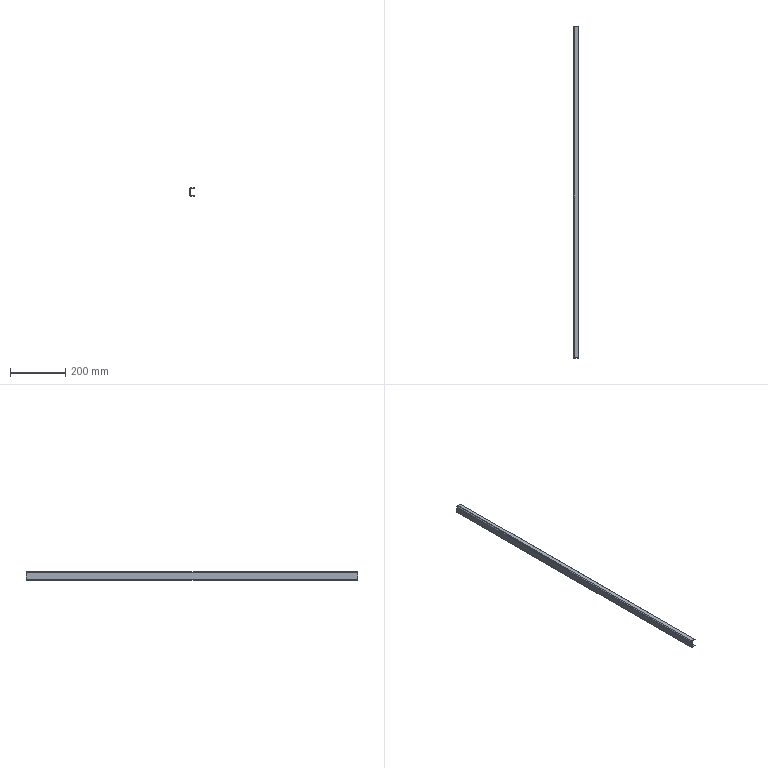Component | SolidWorks | MiddleTopCoverAssembly-1_TopCoverStiffener-1 | 1 solid | 30 faces | box 18 x 1200 x 30 mm | volume 142406 mm3 | plane 26 | cylinder 4 | commonest cylinder face diameters 8 x2 4 x2 | material Plain Carbon Steel
STEP:
#1=CARTESIAN_POINT('',(45.051,0.5334,82.479));
#2=VERTEX_POINT('',#1);
#3=CARTESIAN_POINT('',(45.051,0.5334,82.499));
#4=VERTEX_POINT('',#3);
#5=CARTESIAN_POINT('',(45.051,0.5334,82.42));
#6=DIRECTION('',(-0.,-0.,1.));
#7=VECTOR('',#6,39.37);
#8=LINE('',#5,#7);
#9=EDGE_CURVE('',#2,#4,#8,.T.);
#10=ORIENTED_EDGE('',*,*,#9,.F.);
#11=CARTESIAN_POINT('',(45.051,0.6201,82.479));
#12=VERTEX_POINT('',#11);
#13=CARTESIAN_POINT('',(45.051,47.778,82.479));
#14=DIRECTION('',(0.,1.,0.));
#15=VECTOR('',#14,39.37);
#16=LINE('',#13,#15);
#17=EDGE_CURVE('',#2,#12,#16,.T.);
#18=ORIENTED_EDGE('',*,*,#17,.T.);
#19=CARTESIAN_POINT('',(45.051,0.6201,82.42));
#20=VERTEX_POINT('',#19);
#21=CARTESIAN_POINT('',(45.051,0.6201,82.42));
#22=DIRECTION('',(0.,0.,-1.));
#23=VECTOR('',#22,39.37);
#24=LINE('',#21,#23);
#25=EDGE_CURVE('',#12,#20,#24,.T.);
#26=ORIENTED_EDGE('',*,*,#25,.T.);
#27=CARTESIAN_POINT('',(45.051,47.691,82.42));
#28=VERTEX_POINT('',#27);
#29=CARTESIAN_POINT('',(45.051,47.778,82.42));
#30=DIRECTION('',(-0.,-1.,-0.));
#31=VECTOR('',#30,39.37);
#32=LINE('',#29,#31);
#33=EDGE_CURVE('',#28,#20,#32,.T.);
#34=ORIENTED_EDGE('',*,*,#33,.F.);
#35=CARTESIAN_POINT('',(45.051,47.691,82.479));
#36=VERTEX_POINT('',#35);
#37=CARTESIAN_POINT('',(45.051,47.691,82.42));
#38=DIRECTION('',(-0.,-0.,1.));
#39=VECTOR('',#38,39.37);
#40=LINE('',#37,#39);
#41=EDGE_CURVE('',#28,#36,#40,.T.);
#42=ORIENTED_EDGE('',*,*,#41,.T.);
#43=CARTESIAN_POINT('',(45.051,47.778,82.479));
#44=VERTEX_POINT('',#43);
#45=CARTESIAN_POINT('',(45.051,47.778,82.479));
#46=DIRECTION('',(0.,1.,0.));
#47=VECTOR('',#46,39.37);
#48=LINE('',#45,#47);
#49=EDGE_CURVE('',#36,#44,#48,.T.);
#50=ORIENTED_EDGE('',*,*,#49,.T.);
#51=CARTESIAN_POINT('',(45.051,47.778,82.499));
#52=VERTEX_POINT('',#51);
#53=CARTESIAN_POINT('',(45.051,47.778,82.42));
#54=DIRECTION('',(-0.,-0.,1.));
#55=VECTOR('',#54,39.37);
#56=LINE('',#53,#55);
#57=EDGE_CURVE('',#44,#52,#56,.T.);
#58=ORIENTED_EDGE('',*,*,#57,.T.);
#59=CARTESIAN_POINT('',(45.051,47.778,82.499));
#60=DIRECTION('',(-0.,-1.,-0.));
#61=VECTOR('',#60,39.37);
#62=LINE('',#59,#61);
#63=EDGE_CURVE('',#52,#4,#62,.T.);
#64=ORIENTED_EDGE('',*,*,#63,.T.);
#65=EDGE_LOOP('',(#10,#18,#26,#34,#42,#50,#58,#64));
#66=FACE_OUTER_BOUND('',#65,.T.);
#67=CARTESIAN_POINT('',(45.051,47.778,82.42));
#68=DIRECTION('',(1.,-0.,-0.));
#69=DIRECTION('',(0.,0.,-1.));
#70=AXIS2_PLACEMENT_3D('',#67,#68,#69);
#71=PLANE('',#70);
#72=ADVANCED_FACE('',(#66),#71,.T.);
#73=CARTESIAN_POINT('',(45.051,0.6201,83.602));
#74=VERTEX_POINT('',#73);
#75=CARTESIAN_POINT('',(45.051,0.6201,83.543));
#76=VERTEX_POINT('',#75);
#77=CARTESIAN_POINT('',(45.051,0.6201,83.523));
#78=DIRECTION('',(0.,0.,-1.));
#79=VECTOR('',#78,39.37);
#80=LINE('',#77,#79);
#81=EDGE_CURVE('',#74,#76,#80,.T.);
#82=ORIENTED_EDGE('',*,*,#81,.T.);
#83=CARTESIAN_POINT('',(45.051,0.5334,83.543));
#84=VERTEX_POINT('',#83);
#85=CARTESIAN_POINT('',(45.051,47.778,83.543));
#86=DIRECTION('',(-0.,-1.,-0.));
#87=VECTOR('',#86,39.37);
#88=LINE('',#85,#87);
#89=EDGE_CURVE('',#76,#84,#88,.T.);
#90=ORIENTED_EDGE('',*,*,#89,.T.);
#91=CARTESIAN_POINT('',(45.051,0.5334,83.523));
#92=VERTEX_POINT('',#91);
#93=CARTESIAN_POINT('',(45.051,0.5334,83.523));
#94=DIRECTION('',(-0.,-0.,1.));
#95=VECTOR('',#94,39.37);
#96=LINE('',#93,#95);
#97=EDGE_CURVE('',#92,#84,#96,.T.);
#98=ORIENTED_EDGE('',*,*,#97,.F.);
#99=CARTESIAN_POINT('',(45.051,47.778,83.523));
#100=VERTEX_POINT('',#99);
#101=CARTESIAN_POINT('',(45.051,47.778,83.523));
#102=DIRECTION('',(-0.,-1.,-0.));
#103=VECTOR('',#102,39.37);
#104=LINE('',#101,#103);
#105=EDGE_CURVE('',#100,#92,#104,.T.);
#106=ORIENTED_EDGE('',*,*,#105,.F.);
#107=CARTESIAN_POINT('',(45.051,47.778,83.543));
#108=VERTEX_POINT('',#107);
#109=CARTESIAN_POINT('',(45.051,47.778,83.523));
#110=DIRECTION('',(-0.,-0.,1.));
#111=VECTOR('',#110,39.37);
#112=LINE('',#109,#111);
#113=EDGE_CURVE('',#100,#108,#112,.T.);
#114=ORIENTED_EDGE('',*,*,#113,.T.);
#115=CARTESIAN_POINT('',(45.051,47.691,83.543));
#116=VERTEX_POINT('',#115);
#117=CARTESIAN_POINT('',(45.051,47.778,83.543));
#118=DIRECTION('',(-0.,-1.,-0.));
#119=VECTOR('',#118,39.37);
#120=LINE('',#117,#119);
#121=EDGE_CURVE('',#108,#116,#120,.T.);
#122=ORIENTED_EDGE('',*,*,#121,.T.);
#123=CARTESIAN_POINT('',(45.051,47.691,83.602));
#124=VERTEX_POINT('',#123);
#125=CARTESIAN_POINT('',(45.051,47.691,83.523));
#126=DIRECTION('',(-0.,-0.,1.));
#127=VECTOR('',#126,39.37);
#128=LINE('',#125,#127);
#129=EDGE_CURVE('',#116,#124,#128,.T.);
#130=ORIENTED_EDGE('',*,*,#129,.T.);
#131=CARTESIAN_POINT('',(45.051,47.778,83.602));
#132=DIRECTION('',(-0.,-1.,-0.));
#133=VECTOR('',#132,39.37);
#134=LINE('',#131,#133);
#135=EDGE_CURVE('',#124,#74,#134,.T.);
#136=ORIENTED_EDGE('',*,*,#135,.T.);
#137=EDGE_LOOP('',(#82,#90,#98,#106,#114,#122,#130,#136));
#138=FACE_OUTER_BOUND('',#137,.T.);
#139=CARTESIAN_POINT('',(45.051,47.778,83.523));
#140=DIRECTION('',(1.,-0.,-0.));
#141=DIRECTION('',(-0.,-1.,-0.));
#142=AXIS2_PLACEMENT_3D('',#139,#140,#141);
#143=PLANE('',#142);
#144=ADVANCED_FACE('',(#138),#143,.T.);
#145=CARTESIAN_POINT('',(44.499,47.778,83.543));
#146=VERTEX_POINT('',#145);
#147=CARTESIAN_POINT('',(44.377,47.778,83.543));
#148=VERTEX_POINT('',#147);
#149=CARTESIAN_POINT('',(44.342,47.778,83.543));
#150=DIRECTION('',(-1.,0.,0.));
#151=VECTOR('',#150,39.37);
#152=LINE('',#149,#151);
#153=EDGE_CURVE('',#146,#148,#152,.T.);
#154=ORIENTED_EDGE('',*,*,#153,.F.);
#155=CARTESIAN_POINT('',(44.499,47.778,83.523));
#156=VERTEX_POINT('',#155);
#157=CARTESIAN_POINT('',(44.499,47.778,83.523));
#158=DIRECTION('',(-0.,-0.,1.));
#159=VECTOR('',#158,39.37);
#160=LINE('',#157,#159);
#161=EDGE_CURVE('',#156,#146,#160,.T.);
#162=ORIENTED_EDGE('',*,*,#161,.F.);
#163=CARTESIAN_POINT('',(44.421,47.778,83.444));
#164=VERTEX_POINT('',#163);
#165=CARTESIAN_POINT('',(44.499,47.778,83.444));
#166=DIRECTION('',(-0.,-1.,-0.));
#167=DIRECTION('',(0.,0.,-1.));
#168=AXIS2_PLACEMENT_3D('',#165,#166,#167);
#169=CIRCLE('',#168,0.07874);
#170=EDGE_CURVE('',#156,#164,#169,.T.);
#171=ORIENTED_EDGE('',*,*,#170,.T.);
#172=CARTESIAN_POINT('',(44.342,47.778,83.444));
#173=VERTEX_POINT('',#172);
#174=CARTESIAN_POINT('',(44.342,47.778,83.444));
#175=DIRECTION('',(1.,-0.,-0.));
#176=VECTOR('',#175,39.37);
#177=LINE('',#174,#176);
#178=EDGE_CURVE('',#173,#164,#177,.T.);
#179=ORIENTED_EDGE('',*,*,#178,.F.);
#180=CARTESIAN_POINT('',(44.499,47.778,83.444));
#181=DIRECTION('',(-0.,-1.,-0.));
#182=DIRECTION('',(0.,0.,-1.));
#183=AXIS2_PLACEMENT_3D('',#180,#181,#182);
#184=CIRCLE('',#183,0.1575);
#185=EDGE_CURVE('',#148,#173,#184,.T.);
#186=ORIENTED_EDGE('',*,*,#185,.F.);
#187=EDGE_LOOP('',(#154,#162,#171,#179,#186));
#188=FACE_OUTER_BOUND('',#187,.T.);
#189=CARTESIAN_POINT('',(44.342,47.778,83.444));
#190=DIRECTION('',(0.,1.,0.));
#191=DIRECTION('',(0.,0.,-1.));
#192=AXIS2_PLACEMENT_3D('',#189,#190,#191);
#193=PLANE('',#192);
#194=ADVANCED_FACE('',(#188),#193,.T.);
#195=CARTESIAN_POINT('',(44.342,47.778,82.578));
#196=VERTEX_POINT('',#195);
#197=CARTESIAN_POINT('',(44.342,47.778,83.602));
#198=DIRECTION('',(0.,0.,-1.));
#199=VECTOR('',#198,39.37);
#200=LINE('',#197,#199);
#201=EDGE_CURVE('',#173,#196,#200,.T.);
#202=ORIENTED_EDGE('',*,*,#201,.F.);
#203=ORIENTED_EDGE('',*,*,#178,.T.);
#204=CARTESIAN_POINT('',(44.421,47.778,82.578));
#205=VERTEX_POINT('',#204);
#206=CARTESIAN_POINT('',(44.421,47.778,83.602));
#207=DIRECTION('',(0.,0.,-1.));
#208=VECTOR('',#207,39.37);
#209=LINE('',#206,#208);
#210=EDGE_CURVE('',#164,#205,#209,.T.);
#211=ORIENTED_EDGE('',*,*,#210,.T.);
#212=CARTESIAN_POINT('',(44.421,47.778,82.578));
#213=DIRECTION('',(-1.,0.,0.));
#214=VECTOR('',#213,39.37);
#215=LINE('',#212,#214);
#216=EDGE_CURVE('',#205,#196,#215,.T.);
#217=ORIENTED_EDGE('',*,*,#216,.T.);
#218=EDGE_LOOP('',(#202,#203,#211,#217));
#219=FACE_OUTER_BOUND('',#218,.T.);
#220=CARTESIAN_POINT('',(44.499,47.778,83.523));
#221=DIRECTION('',(0.,1.,0.));
#222=DIRECTION('',(0.,0.,-1.));
#223=AXIS2_PLACEMENT_3D('',#220,#221,#222);
#224=PLANE('',#223);
#225=ADVANCED_FACE('',(#219),#224,.T.);
#226=CARTESIAN_POINT('',(44.377,0.5334,83.543));
#227=VERTEX_POINT('',#226);
#228=CARTESIAN_POINT('',(44.499,0.5334,83.543));
#229=VERTEX_POINT('',#228);
#230=CARTESIAN_POINT('',(44.499,0.5334,83.543));
#231=DIRECTION('',(1.,-0.,-0.));
#232=VECTOR('',#231,39.37);
#233=LINE('',#230,#232);
#234=EDGE_CURVE('',#227,#229,#233,.T.);
#235=ORIENTED_EDGE('',*,*,#234,.F.);
#236=CARTESIAN_POINT('',(44.342,0.5334,83.444));
#237=VERTEX_POINT('',#236);
#238=CARTESIAN_POINT('',(44.499,0.5334,83.444));
#239=DIRECTION('',(-0.,-1.,-0.));
#240=DIRECTION('',(0.,0.,-1.));
#241=AXIS2_PLACEMENT_3D('',#238,#239,#240);
#242=CIRCLE('',#241,0.1575);
#243=EDGE_CURVE('',#227,#237,#242,.T.);
#244=ORIENTED_EDGE('',*,*,#243,.T.);
#245=CARTESIAN_POINT('',(44.421,0.5334,83.444));
#246=VERTEX_POINT('',#245);
#247=CARTESIAN_POINT('',(44.421,0.5334,83.444));
#248=DIRECTION('',(-1.,0.,0.));
#249=VECTOR('',#248,39.37);
#250=LINE('',#247,#249);
#251=EDGE_CURVE('',#246,#237,#250,.T.);
#252=ORIENTED_EDGE('',*,*,#251,.F.);
#253=CARTESIAN_POINT('',(44.499,0.5334,83.523));
#254=VERTEX_POINT('',#253);
#255=CARTESIAN_POINT('',(44.499,0.5334,83.444));
#256=DIRECTION('',(-0.,-1.,-0.));
#257=DIRECTION('',(0.,0.,-1.));
#258=AXIS2_PLACEMENT_3D('',#255,#256,#257);
#259=CIRCLE('',#258,0.07874);
#260=EDGE_CURVE('',#254,#246,#259,.T.);
#261=ORIENTED_EDGE('',*,*,#260,.F.);
#262=CARTESIAN_POINT('',(44.499,0.5334,83.602));
#263=DIRECTION('',(0.,0.,-1.));
#264=VECTOR('',#263,39.37);
#265=LINE('',#262,#264);
#266=EDGE_CURVE('',#229,#254,#265,.T.);
#267=ORIENTED_EDGE('',*,*,#266,.F.);
#268=EDGE_LOOP('',(#235,#244,#252,#261,#267));
#269=FACE_OUTER_BOUND('',#268,.T.);
#270=CARTESIAN_POINT('',(44.499,0.5334,83.602));
#271=DIRECTION('',(-0.,-1.,-0.));
#272=DIRECTION('',(-0.,-0.,1.));
#273=AXIS2_PLACEMENT_3D('',#270,#271,#272);
#274=PLANE('',#273);
#275=ADVANCED_FACE('',(#269),#274,.T.);
#276=CARTESIAN_POINT('',(44.421,0.5334,83.543));
#277=DIRECTION('',(1.,-0.,-0.));
#278=VECTOR('',#277,39.37);
#279=LINE('',#276,#278);
#280=EDGE_CURVE('',#229,#84,#279,.T.);
#281=ORIENTED_EDGE('',*,*,#280,.F.);
#282=ORIENTED_EDGE('',*,*,#266,.T.);
#283=CARTESIAN_POINT('',(45.051,0.5334,83.523));
#284=DIRECTION('',(-1.,0.,0.));
#285=VECTOR('',#284,39.37);
#286=LINE('',#283,#285);
#287=EDGE_CURVE('',#92,#254,#286,.T.);
#288=ORIENTED_EDGE('',*,*,#287,.F.);
#289=ORIENTED_EDGE('',*,*,#97,.T.);
#290=EDGE_LOOP('',(#281,#282,#288,#289));
#291=FACE_OUTER_BOUND('',#290,.T.);
#292=CARTESIAN_POINT('',(44.421,0.5334,83.444));
#293=DIRECTION('',(-0.,-1.,-0.));
#294=DIRECTION('',(-0.,-0.,1.));
#295=AXIS2_PLACEMENT_3D('',#292,#293,#294);
#296=PLANE('',#295);
#297=ADVANCED_FACE('',(#291),#296,.T.);
#298=CARTESIAN_POINT('',(44.377,47.778,82.479));
#299=VERTEX_POINT('',#298);
#300=CARTESIAN_POINT('',(44.499,47.778,82.479));
#301=VERTEX_POINT('',#300);
#302=CARTESIAN_POINT('',(44.499,47.778,82.479));
#303=DIRECTION('',(1.,-0.,-0.));
#304=VECTOR('',#303,39.37);
#305=LINE('',#302,#304);
#306=EDGE_CURVE('',#299,#301,#305,.T.);
#307=ORIENTED_EDGE('',*,*,#306,.F.);
#308=CARTESIAN_POINT('',(44.499,47.778,82.578));
#309=DIRECTION('',(-0.,-1.,-0.));
#310=DIRECTION('',(0.,0.,-1.));
#311=AXIS2_PLACEMENT_3D('',#308,#309,#310);
#312=CIRCLE('',#311,0.1575);
#313=EDGE_CURVE('',#196,#299,#312,.T.);
#314=ORIENTED_EDGE('',*,*,#313,.F.);
#315=ORIENTED_EDGE('',*,*,#216,.F.);
#316=CARTESIAN_POINT('',(44.499,47.778,82.499));
#317=VERTEX_POINT('',#316);
#318=CARTESIAN_POINT('',(44.499,47.778,82.578));
#319=DIRECTION('',(-0.,-1.,-0.));
#320=DIRECTION('',(0.,0.,-1.));
#321=AXIS2_PLACEMENT_3D('',#318,#319,#320);
#322=CIRCLE('',#321,0.07874);
#323=EDGE_CURVE('',#205,#317,#322,.T.);
#324=ORIENTED_EDGE('',*,*,#323,.T.);
#325=CARTESIAN_POINT('',(44.499,47.778,82.42));
#326=DIRECTION('',(-0.,-0.,1.));
#327=VECTOR('',#326,39.37);
#328=LINE('',#325,#327);
#329=EDGE_CURVE('',#301,#317,#328,.T.);
#330=ORIENTED_EDGE('',*,*,#329,.F.);
#331=EDGE_LOOP('',(#307,#314,#315,#324,#330));
#332=FACE_OUTER_BOUND('',#331,.T.);
#333=CARTESIAN_POINT('',(44.499,47.778,82.42));
#334=DIRECTION('',(0.,1.,0.));
#335=DIRECTION('',(0.,0.,-1.));
#336=AXIS2_PLACEMENT_3D('',#333,#334,#335);
#337=PLANE('',#336);
#338=ADVANCED_FACE('',(#332),#337,.T.);
#339=CARTESIAN_POINT('',(44.421,47.778,82.479));
#340=DIRECTION('',(1.,-0.,-0.));
#341=VECTOR('',#340,39.37);
#342=LINE('',#339,#341);
#343=EDGE_CURVE('',#301,#44,#342,.T.);
#344=ORIENTED_EDGE('',*,*,#343,.F.);
#345=ORIENTED_EDGE('',*,*,#329,.T.);
#346=CARTESIAN_POINT('',(44.342,47.778,82.499));
#347=DIRECTION('',(1.,-0.,-0.));
#348=VECTOR('',#347,39.37);
#349=LINE('',#346,#348);
#350=EDGE_CURVE('',#317,#52,#349,.T.);
#351=ORIENTED_EDGE('',*,*,#350,.T.);
#352=ORIENTED_EDGE('',*,*,#57,.F.);
#353=EDGE_LOOP('',(#344,#345,#351,#352));
#354=FACE_OUTER_BOUND('',#353,.T.);
#355=CARTESIAN_POINT('',(44.421,47.778,82.578));
#356=DIRECTION('',(0.,1.,0.));
#357=DIRECTION('',(0.,0.,-1.));
#358=AXIS2_PLACEMENT_3D('',#355,#356,#357);
#359=PLANE('',#358);
#360=ADVANCED_FACE('',(#354),#359,.T.);
#361=CARTESIAN_POINT('',(44.499,0.5334,82.479));
#362=VERTEX_POINT('',#361);
#363=CARTESIAN_POINT('',(44.377,0.5334,82.479));
#364=VERTEX_POINT('',#363);
#365=CARTESIAN_POINT('',(44.342,0.5334,82.479));
#366=DIRECTION('',(-1.,0.,0.));
#367=VECTOR('',#366,39.37);
#368=LINE('',#365,#367);
#369=EDGE_CURVE('',#362,#364,#368,.T.);
#370=ORIENTED_EDGE('',*,*,#369,.F.);
#371=CARTESIAN_POINT('',(44.499,0.5334,82.499));
#372=VERTEX_POINT('',#371);
#373=CARTESIAN_POINT('',(44.499,0.5334,82.499));
#374=DIRECTION('',(0.,0.,-1.));
#375=VECTOR('',#374,39.37);
#376=LINE('',#373,#375);
#377=EDGE_CURVE('',#372,#362,#376,.T.);
#378=ORIENTED_EDGE('',*,*,#377,.F.);
#379=CARTESIAN_POINT('',(44.421,0.5334,82.578));
#380=VERTEX_POINT('',#379);
#381=CARTESIAN_POINT('',(44.499,0.5334,82.578));
#382=DIRECTION('',(-0.,-1.,-0.));
#383=DIRECTION('',(0.,0.,-1.));
#384=AXIS2_PLACEMENT_3D('',#381,#382,#383);
#385=CIRCLE('',#384,0.07874);
#386=EDGE_CURVE('',#380,#372,#385,.T.);
#387=ORIENTED_EDGE('',*,*,#386,.F.);
#388=CARTESIAN_POINT('',(44.342,0.5334,82.578));
#389=VERTEX_POINT('',#388);
#390=CARTESIAN_POINT('',(44.342,0.5334,82.578));
#391=DIRECTION('',(1.,-0.,-0.));
#392=VECTOR('',#391,39.37);
#393=LINE('',#390,#392);
#394=EDGE_CURVE('',#389,#380,#393,.T.);
#395=ORIENTED_EDGE('',*,*,#394,.F.);
#396=CARTESIAN_POINT('',(44.499,0.5334,82.578));
#397=DIRECTION('',(-0.,-1.,-0.));
#398=DIRECTION('',(0.,0.,-1.));
#399=AXIS2_PLACEMENT_3D('',#396,#397,#398);
#400=CIRCLE('',#399,0.1575);
#401=EDGE_CURVE('',#389,#364,#400,.T.);
#402=ORIENTED_EDGE('',*,*,#401,.T.);
#403=EDGE_LOOP('',(#370,#378,#387,#395,#402));
#404=FACE_OUTER_BOUND('',#403,.T.);
#405=CARTESIAN_POINT('',(44.342,0.5334,82.578));
#406=DIRECTION('',(-0.,-1.,-0.));
#407=DIRECTION('',(-0.,-0.,1.));
#408=AXIS2_PLACEMENT_3D('',#405,#406,#407);
#409=PLANE('',#408);
#410=ADVANCED_FACE('',(#404),#409,.T.);
#411=CARTESIAN_POINT('',(44.342,0.5334,83.602));
#412=DIRECTION('',(0.,0.,-1.));
#413=VECTOR('',#412,39.37);
#414=LINE('',#411,#413);
#415=EDGE_CURVE('',#237,#389,#414,.T.);
#416=ORIENTED_EDGE('',*,*,#415,.T.);
#417=ORIENTED_EDGE('',*,*,#394,.T.);
#418=CARTESIAN_POINT('',(44.421,0.5334,83.602));
#419=DIRECTION('',(0.,0.,-1.));
#420=VECTOR('',#419,39.37);
#421=LINE('',#418,#420);
#422=EDGE_CURVE('',#246,#380,#421,.T.);
#423=ORIENTED_EDGE('',*,*,#422,.F.);
#424=ORIENTED_EDGE('',*,*,#251,.T.);
#425=EDGE_LOOP('',(#416,#417,#423,#424));
#426=FACE_OUTER_BOUND('',#425,.T.);
#427=CARTESIAN_POINT('',(44.499,0.5334,82.499));
#428=DIRECTION('',(-0.,-1.,-0.));
#429=DIRECTION('',(-0.,-0.,1.));
#430=AXIS2_PLACEMENT_3D('',#427,#428,#429);
#431=PLANE('',#430);
#432=ADVANCED_FACE('',(#426),#431,.T.);
#433=CARTESIAN_POINT('',(44.342,0.5334,82.499));
#434=DIRECTION('',(1.,-0.,-0.));
#435=VECTOR('',#434,39.37);
#436=LINE('',#433,#435);
#437=EDGE_CURVE('',#372,#4,#436,.T.);
#438=ORIENTED_EDGE('',*,*,#437,.T.);
#439=ORIENTED_EDGE('',*,*,#63,.F.);
#440=ORIENTED_EDGE('',*,*,#350,.F.);
#441=CARTESIAN_POINT('',(44.499,47.778,82.499));
#442=DIRECTION('',(-0.,-1.,-0.));
#443=VECTOR('',#442,39.37);
#444=LINE('',#441,#443);
#445=EDGE_CURVE('',#317,#372,#444,.T.);
#446=ORIENTED_EDGE('',*,*,#445,.T.);
#447=EDGE_LOOP('',(#438,#439,#440,#446));
#448=FACE_OUTER_BOUND('',#447,.T.);
#449=CARTESIAN_POINT('',(44.342,47.778,82.499));
#450=DIRECTION('',(-0.,0.,-1.));
#451=DIRECTION('',(-1.,0.,0.));
#452=AXIS2_PLACEMENT_3D('',#449,#450,#451);
#453=PLANE('',#452);
#454=ADVANCED_FACE('',(#448),#453,.F.);
#455=CARTESIAN_POINT('',(44.499,0.6201,82.42));
#456=VERTEX_POINT('',#455);
#457=CARTESIAN_POINT('',(44.342,0.6201,82.42));
#458=DIRECTION('',(1.,-0.,-0.));
#459=VECTOR('',#458,39.37);
#460=LINE('',#457,#459);
#461=EDGE_CURVE('',#456,#20,#460,.T.);
#462=ORIENTED_EDGE('',*,*,#461,.F.);
#463=CARTESIAN_POINT('',(44.499,47.691,82.42));
#464=VERTEX_POINT('',#463);
#465=CARTESIAN_POINT('',(44.499,47.778,82.42));
#466=DIRECTION('',(-0.,-1.,-0.));
#467=VECTOR('',#466,39.37);
#468=LINE('',#465,#467);
#469=EDGE_CURVE('',#464,#456,#468,.T.);
#470=ORIENTED_EDGE('',*,*,#469,.F.);
#471=CARTESIAN_POINT('',(44.342,47.691,82.42));
#472=DIRECTION('',(-1.,0.,0.));
#473=VECTOR('',#472,39.37);
#474=LINE('',#471,#473);
#475=EDGE_CURVE('',#28,#464,#474,.T.);
#476=ORIENTED_EDGE('',*,*,#475,.F.);
#477=ORIENTED_EDGE('',*,*,#33,.T.);
#478=EDGE_LOOP('',(#462,#470,#476,#477));
#479=FACE_OUTER_BOUND('',#478,.T.);
#480=CARTESIAN_POINT('',(44.342,47.778,82.42));
#481=DIRECTION('',(-0.,0.,-1.));
#482=DIRECTION('',(-1.,0.,0.));
#483=AXIS2_PLACEMENT_3D('',#480,#481,#482);
#484=PLANE('',#483);
#485=ADVANCED_FACE('',(#479),#484,.T.);
#486=CARTESIAN_POINT('',(44.377,0.6201,82.479));
#487=VERTEX_POINT('',#486);
#488=CARTESIAN_POINT('',(44.377,47.778,82.479));
#489=DIRECTION('',(0.,1.,0.));
#490=VECTOR('',#489,39.37);
#491=LINE('',#488,#490);
#492=EDGE_CURVE('',#364,#487,#491,.T.);
#493=ORIENTED_EDGE('',*,*,#492,.F.);
#494=ORIENTED_EDGE('',*,*,#401,.F.);
#495=CARTESIAN_POINT('',(44.342,47.778,82.578));
#496=DIRECTION('',(-0.,-1.,-0.));
#497=VECTOR('',#496,39.37);
#498=LINE('',#495,#497);
#499=EDGE_CURVE('',#196,#389,#498,.T.);
#500=ORIENTED_EDGE('',*,*,#499,.F.);
#501=ORIENTED_EDGE('',*,*,#313,.T.);
#502=CARTESIAN_POINT('',(44.377,47.691,82.479));
#503=VERTEX_POINT('',#502);
#504=CARTESIAN_POINT('',(44.377,47.778,82.479));
#505=DIRECTION('',(0.,1.,0.));
#506=VECTOR('',#505,39.37);
#507=LINE('',#504,#506);
#508=EDGE_CURVE('',#503,#299,#507,.T.);
#509=ORIENTED_EDGE('',*,*,#508,.F.);
#510=CARTESIAN_POINT('',(44.499,47.691,82.578));
#511=DIRECTION('',(0.,1.,0.));
#512=DIRECTION('',(-0.,0.,1.));
#513=AXIS2_PLACEMENT_3D('',#510,#511,#512);
#514=CIRCLE('',#513,0.1575);
#515=EDGE_CURVE('',#464,#503,#514,.T.);
#516=ORIENTED_EDGE('',*,*,#515,.F.);
#517=ORIENTED_EDGE('',*,*,#469,.T.);
#518=CARTESIAN_POINT('',(44.499,0.6201,82.578));
#519=DIRECTION('',(-0.,-1.,-0.));
#520=DIRECTION('',(-0.,0.,-1.));
#521=AXIS2_PLACEMENT_3D('',#518,#519,#520);
#522=CIRCLE('',#521,0.1575);
#523=EDGE_CURVE('',#487,#456,#522,.T.);
#524=ORIENTED_EDGE('',*,*,#523,.F.);
#525=EDGE_LOOP('',(#493,#494,#500,#501,#509,#516,#517,#524));
#526=FACE_OUTER_BOUND('',#525,.T.);
#527=CARTESIAN_POINT('',(44.499,47.778,82.578));
#528=DIRECTION('',(-0.,-1.,-0.));
#529=DIRECTION('',(0.,0.,1.));
#530=AXIS2_PLACEMENT_3D('',#527,#528,#529);
#531=CYLINDRICAL_SURFACE('',#530,0.1575);
#532=ADVANCED_FACE('',(#526),#531,.T.);
#533=ORIENTED_EDGE('',*,*,#415,.F.);
#534=CARTESIAN_POINT('',(44.342,47.778,83.444));
#535=DIRECTION('',(-0.,-1.,-0.));
#536=VECTOR('',#535,39.37);
#537=LINE('',#534,#536);
#538=EDGE_CURVE('',#173,#237,#537,.T.);
#539=ORIENTED_EDGE('',*,*,#538,.F.);
#540=ORIENTED_EDGE('',*,*,#201,.T.);
#541=ORIENTED_EDGE('',*,*,#499,.T.);
#542=EDGE_LOOP('',(#533,#539,#540,#541));
#543=FACE_OUTER_BOUND('',#542,.T.);
#544=CARTESIAN_POINT('',(44.342,47.778,83.602));
#545=DIRECTION('',(-1.,0.,0.));
#546=DIRECTION('',(0.,1.,0.));
#547=AXIS2_PLACEMENT_3D('',#544,#545,#546);
#548=PLANE('',#547);
#549=ADVANCED_FACE('',(#543),#548,.T.);
#550=CARTESIAN_POINT('',(44.377,0.6201,83.543));
#551=VERTEX_POINT('',#550);
#552=CARTESIAN_POINT('',(44.377,47.778,83.543));
#553=DIRECTION('',(-0.,-1.,-0.));
#554=VECTOR('',#553,39.37);
#555=LINE('',#552,#554);
#556=EDGE_CURVE('',#551,#227,#555,.T.);
#557=ORIENTED_EDGE('',*,*,#556,.F.);
#558=CARTESIAN_POINT('',(44.499,0.6201,83.602));
#559=VERTEX_POINT('',#558);
#560=CARTESIAN_POINT('',(44.499,0.6201,83.444));
#561=DIRECTION('',(-0.,-1.,-0.));
#562=DIRECTION('',(0.,0.,-1.));
#563=AXIS2_PLACEMENT_3D('',#560,#561,#562);
#564=CIRCLE('',#563,0.1575);
#565=EDGE_CURVE('',#559,#551,#564,.T.);
#566=ORIENTED_EDGE('',*,*,#565,.F.);
#567=CARTESIAN_POINT('',(44.499,47.691,83.602));
#568=VERTEX_POINT('',#567);
#569=CARTESIAN_POINT('',(44.499,47.778,83.602));
#570=DIRECTION('',(-0.,-1.,-0.));
#571=VECTOR('',#570,39.37);
#572=LINE('',#569,#571);
#573=EDGE_CURVE('',#568,#559,#572,.T.);
#574=ORIENTED_EDGE('',*,*,#573,.F.);
#575=CARTESIAN_POINT('',(44.377,47.691,83.543));
#576=VERTEX_POINT('',#575);
#577=CARTESIAN_POINT('',(44.499,47.691,83.444));
#578=DIRECTION('',(0.,1.,0.));
#579=DIRECTION('',(0.,0.,1.));
#580=AXIS2_PLACEMENT_3D('',#577,#578,#579);
#581=CIRCLE('',#580,0.1575);
#582=EDGE_CURVE('',#576,#568,#581,.T.);
#583=ORIENTED_EDGE('',*,*,#582,.F.);
#584=CARTESIAN_POINT('',(44.377,47.778,83.543));
#585=DIRECTION('',(-0.,-1.,-0.));
#586=VECTOR('',#585,39.37);
#587=LINE('',#584,#586);
#588=EDGE_CURVE('',#148,#576,#587,.T.);
#589=ORIENTED_EDGE('',*,*,#588,.F.);
#590=ORIENTED_EDGE('',*,*,#185,.T.);
#591=ORIENTED_EDGE('',*,*,#538,.T.);
#592=ORIENTED_EDGE('',*,*,#243,.F.);
#593=EDGE_LOOP('',(#557,#566,#574,#583,#589,#590,#591,#592));
#594=FACE_OUTER_BOUND('',#593,.T.);
#595=CARTESIAN_POINT('',(44.499,47.778,83.444));
#596=DIRECTION('',(-0.,-1.,-0.));
#597=DIRECTION('',(0.,0.,1.));
#598=AXIS2_PLACEMENT_3D('',#595,#596,#597);
#599=CYLINDRICAL_SURFACE('',#598,0.1575);
#600=ADVANCED_FACE('',(#594),#599,.T.);
#601=CARTESIAN_POINT('',(45.051,0.6201,83.602));
#602=DIRECTION('',(-1.,0.,0.));
#603=VECTOR('',#602,39.37);
#604=LINE('',#601,#603);
#605=EDGE_CURVE('',#74,#559,#604,.T.);
#606=ORIENTED_EDGE('',*,*,#605,.F.);
#607=ORIENTED_EDGE('',*,*,#135,.F.);
#608=CARTESIAN_POINT('',(45.051,47.691,83.602));
#609=DIRECTION('',(1.,-0.,-0.));
#610=VECTOR('',#609,39.37);
#611=LINE('',#608,#610);
#612=EDGE_CURVE('',#568,#124,#611,.T.);
#613=ORIENTED_EDGE('',*,*,#612,.F.);
#614=ORIENTED_EDGE('',*,*,#573,.T.);
#615=EDGE_LOOP('',(#606,#607,#613,#614));
#616=FACE_OUTER_BOUND('',#615,.T.);
#617=CARTESIAN_POINT('',(45.051,47.778,83.602));
#618=DIRECTION('',(-0.,-0.,1.));
#619=DIRECTION('',(0.,1.,0.));
#620=AXIS2_PLACEMENT_3D('',#617,#618,#619);
#621=PLANE('',#620);
#622=ADVANCED_FACE('',(#616),#621,.T.);
#623=ORIENTED_EDGE('',*,*,#287,.T.);
#624=CARTESIAN_POINT('',(44.499,47.778,83.523));
#625=DIRECTION('',(-0.,-1.,-0.));
#626=VECTOR('',#625,39.37);
#627=LINE('',#624,#626);
#628=EDGE_CURVE('',#156,#254,#627,.T.);
#629=ORIENTED_EDGE('',*,*,#628,.F.);
#630=CARTESIAN_POINT('',(45.051,47.778,83.523));
#631=DIRECTION('',(-1.,0.,0.));
#632=VECTOR('',#631,39.37);
#633=LINE('',#630,#632);
#634=EDGE_CURVE('',#100,#156,#633,.T.);
#635=ORIENTED_EDGE('',*,*,#634,.F.);
#636=ORIENTED_EDGE('',*,*,#105,.T.);
#637=EDGE_LOOP('',(#623,#629,#635,#636));
#638=FACE_OUTER_BOUND('',#637,.T.);
#639=CARTESIAN_POINT('',(45.051,47.778,83.523));
#640=DIRECTION('',(-0.,-0.,1.));
#641=DIRECTION('',(0.,1.,0.));
#642=AXIS2_PLACEMENT_3D('',#639,#640,#641);
#643=PLANE('',#642);
#644=ADVANCED_FACE('',(#638),#643,.F.);
#645=ORIENTED_EDGE('',*,*,#260,.T.);
#646=CARTESIAN_POINT('',(44.421,47.778,83.444));
#647=DIRECTION('',(-0.,-1.,-0.));
#648=VECTOR('',#647,39.37);
#649=LINE('',#646,#648);
#650=EDGE_CURVE('',#164,#246,#649,.T.);
#651=ORIENTED_EDGE('',*,*,#650,.F.);
#652=ORIENTED_EDGE('',*,*,#170,.F.);
#653=ORIENTED_EDGE('',*,*,#628,.T.);
#654=EDGE_LOOP('',(#645,#651,#652,#653));
#655=FACE_OUTER_BOUND('',#654,.T.);
#656=CARTESIAN_POINT('',(44.499,47.778,83.444));
#657=DIRECTION('',(-0.,-1.,-0.));
#658=DIRECTION('',(0.,0.,1.));
#659=AXIS2_PLACEMENT_3D('',#656,#657,#658);
#660=CYLINDRICAL_SURFACE('',#659,0.07874);
#661=ADVANCED_FACE('',(#655),#660,.F.);
#662=ORIENTED_EDGE('',*,*,#422,.T.);
#663=CARTESIAN_POINT('',(44.421,47.778,82.578));
#664=DIRECTION('',(-0.,-1.,-0.));
#665=VECTOR('',#664,39.37);
#666=LINE('',#663,#665);
#667=EDGE_CURVE('',#205,#380,#666,.T.);
#668=ORIENTED_EDGE('',*,*,#667,.F.);
#669=ORIENTED_EDGE('',*,*,#210,.F.);
#670=ORIENTED_EDGE('',*,*,#650,.T.);
#671=EDGE_LOOP('',(#662,#668,#669,#670));
#672=FACE_OUTER_BOUND('',#671,.T.);
#673=CARTESIAN_POINT('',(44.421,47.778,83.602));
#674=DIRECTION('',(-1.,0.,0.));
#675=DIRECTION('',(0.,1.,0.));
#676=AXIS2_PLACEMENT_3D('',#673,#674,#675);
#677=PLANE('',#676);
#678=ADVANCED_FACE('',(#672),#677,.F.);
#679=ORIENTED_EDGE('',*,*,#386,.T.);
#680=ORIENTED_EDGE('',*,*,#445,.F.);
#681=ORIENTED_EDGE('',*,*,#323,.F.);
#682=ORIENTED_EDGE('',*,*,#667,.T.);
#683=EDGE_LOOP('',(#679,#680,#681,#682));
#684=FACE_OUTER_BOUND('',#683,.T.);
#685=CARTESIAN_POINT('',(44.499,47.778,82.578));
#686=DIRECTION('',(-0.,-1.,-0.));
#687=DIRECTION('',(0.,0.,1.));
#688=AXIS2_PLACEMENT_3D('',#685,#686,#687);
#689=CYLINDRICAL_SURFACE('',#688,0.07874);
#690=ADVANCED_FACE('',(#684),#689,.F.);
#691=CARTESIAN_POINT('',(44.499,47.778,83.543));
#692=DIRECTION('',(-1.,0.,0.));
#693=VECTOR('',#692,39.37);
#694=LINE('',#691,#693);
#695=EDGE_CURVE('',#108,#146,#694,.T.);
#696=ORIENTED_EDGE('',*,*,#695,.F.);
#697=ORIENTED_EDGE('',*,*,#113,.F.);
#698=ORIENTED_EDGE('',*,*,#634,.T.);
#699=ORIENTED_EDGE('',*,*,#161,.T.);
#700=EDGE_LOOP('',(#696,#697,#698,#699));
#701=FACE_OUTER_BOUND('',#700,.T.);
#702=CARTESIAN_POINT('',(44.499,47.778,82.578));
#703=DIRECTION('',(0.,1.,0.));
#704=DIRECTION('',(0.,0.,-1.));
#705=AXIS2_PLACEMENT_3D('',#702,#703,#704);
#706=PLANE('',#705);
#707=ADVANCED_FACE('',(#701),#706,.T.);
#708=ORIENTED_EDGE('',*,*,#377,.T.);
#709=CARTESIAN_POINT('',(44.499,0.5334,82.479));
#710=DIRECTION('',(1.,-0.,-0.));
#711=VECTOR('',#710,39.37);
#712=LINE('',#709,#711);
#713=EDGE_CURVE('',#362,#2,#712,.T.);
#714=ORIENTED_EDGE('',*,*,#713,.T.);
#715=ORIENTED_EDGE('',*,*,#9,.T.);
#716=ORIENTED_EDGE('',*,*,#437,.F.);
#717=EDGE_LOOP('',(#708,#714,#715,#716));
#718=FACE_OUTER_BOUND('',#717,.T.);
#719=CARTESIAN_POINT('',(44.499,0.5334,82.578));
#720=DIRECTION('',(0.,1.,0.));
#721=DIRECTION('',(0.,0.,-1.));
#722=AXIS2_PLACEMENT_3D('',#719,#720,#721);
#723=PLANE('',#722);
#724=ADVANCED_FACE('',(#718),#723,.F.);
#725=ORIENTED_EDGE('',*,*,#582,.T.);
#726=ORIENTED_EDGE('',*,*,#612,.T.);
#727=ORIENTED_EDGE('',*,*,#129,.F.);
#728=CARTESIAN_POINT('',(45.051,47.691,83.543));
#729=DIRECTION('',(-1.,0.,0.));
#730=VECTOR('',#729,39.37);
#731=LINE('',#728,#730);
#732=EDGE_CURVE('',#116,#576,#731,.T.);
#733=ORIENTED_EDGE('',*,*,#732,.T.);
#734=EDGE_LOOP('',(#725,#726,#727,#733));
#735=FACE_OUTER_BOUND('',#734,.T.);
#736=CARTESIAN_POINT('',(45.051,47.691,83.63));
#737=DIRECTION('',(-0.,-1.,-0.));
#738=DIRECTION('',(-0.,-0.,1.));
#739=AXIS2_PLACEMENT_3D('',#736,#737,#738);
#740=PLANE('',#739);
#741=ADVANCED_FACE('',(#735),#740,.F.);
#742=ORIENTED_EDGE('',*,*,#588,.T.);
#743=ORIENTED_EDGE('',*,*,#732,.F.);
#744=ORIENTED_EDGE('',*,*,#121,.F.);
#745=ORIENTED_EDGE('',*,*,#695,.T.);
#746=ORIENTED_EDGE('',*,*,#153,.T.);
#747=EDGE_LOOP('',(#742,#743,#744,#745,#746));
#748=FACE_OUTER_BOUND('',#747,.T.);
#749=CARTESIAN_POINT('',(45.051,47.691,83.543));
#750=DIRECTION('',(0.,0.,-1.));
#751=DIRECTION('',(-0.,-1.,-0.));
#752=AXIS2_PLACEMENT_3D('',#749,#750,#751);
#753=PLANE('',#752);
#754=ADVANCED_FACE('',(#748),#753,.F.);
#755=ORIENTED_EDGE('',*,*,#280,.T.);
#756=ORIENTED_EDGE('',*,*,#89,.F.);
#757=CARTESIAN_POINT('',(45.051,0.6201,83.543));
#758=DIRECTION('',(-1.,0.,0.));
#759=VECTOR('',#758,39.37);
#760=LINE('',#757,#759);
#761=EDGE_CURVE('',#76,#551,#760,.T.);
#762=ORIENTED_EDGE('',*,*,#761,.T.);
#763=ORIENTED_EDGE('',*,*,#556,.T.);
#764=ORIENTED_EDGE('',*,*,#234,.T.);
#765=EDGE_LOOP('',(#755,#756,#762,#763,#764));
#766=FACE_OUTER_BOUND('',#765,.T.);
#767=CARTESIAN_POINT('',(45.051,0.5039,83.543));
#768=DIRECTION('',(0.,0.,-1.));
#769=DIRECTION('',(-0.,-1.,-0.));
#770=AXIS2_PLACEMENT_3D('',#767,#768,#769);
#771=PLANE('',#770);
#772=ADVANCED_FACE('',(#766),#771,.F.);
#773=ORIENTED_EDGE('',*,*,#565,.T.);
#774=ORIENTED_EDGE('',*,*,#761,.F.);
#775=ORIENTED_EDGE('',*,*,#81,.F.);
#776=ORIENTED_EDGE('',*,*,#605,.T.);
#777=EDGE_LOOP('',(#773,#774,#775,#776));
#778=FACE_OUTER_BOUND('',#777,.T.);
#779=CARTESIAN_POINT('',(45.051,0.6201,83.63));
#780=DIRECTION('',(0.,1.,0.));
#781=DIRECTION('',(0.,0.,-1.));
#782=AXIS2_PLACEMENT_3D('',#779,#780,#781);
#783=PLANE('',#782);
#784=ADVANCED_FACE('',(#778),#783,.F.);
#785=ORIENTED_EDGE('',*,*,#492,.T.);
#786=CARTESIAN_POINT('',(45.051,0.6201,82.479));
#787=DIRECTION('',(-1.,0.,0.));
#788=VECTOR('',#787,39.37);
#789=LINE('',#786,#788);
#790=EDGE_CURVE('',#12,#487,#789,.T.);
#791=ORIENTED_EDGE('',*,*,#790,.F.);
#792=ORIENTED_EDGE('',*,*,#17,.F.);
#793=ORIENTED_EDGE('',*,*,#713,.F.);
#794=ORIENTED_EDGE('',*,*,#369,.T.);
#795=EDGE_LOOP('',(#785,#791,#792,#793,#794));
#796=FACE_OUTER_BOUND('',#795,.T.);
#797=CARTESIAN_POINT('',(45.051,0.5039,82.479));
#798=DIRECTION('',(-0.,-0.,1.));
#799=DIRECTION('',(0.,1.,0.));
#800=AXIS2_PLACEMENT_3D('',#797,#798,#799);
#801=PLANE('',#800);
#802=ADVANCED_FACE('',(#796),#801,.F.);
#803=ORIENTED_EDGE('',*,*,#461,.T.);
#804=ORIENTED_EDGE('',*,*,#25,.F.);
#805=ORIENTED_EDGE('',*,*,#790,.T.);
#806=ORIENTED_EDGE('',*,*,#523,.T.);
#807=EDGE_LOOP('',(#803,#804,#805,#806));
#808=FACE_OUTER_BOUND('',#807,.T.);
#809=CARTESIAN_POINT('',(45.051,0.6201,82.479));
#810=DIRECTION('',(0.,1.,0.));
#811=DIRECTION('',(0.,0.,-1.));
#812=AXIS2_PLACEMENT_3D('',#809,#810,#811);
#813=PLANE('',#812);
#814=ADVANCED_FACE('',(#808),#813,.F.);
#815=ORIENTED_EDGE('',*,*,#343,.T.);
#816=ORIENTED_EDGE('',*,*,#49,.F.);
#817=CARTESIAN_POINT('',(45.051,47.691,82.479));
#818=DIRECTION('',(-1.,0.,0.));
#819=VECTOR('',#818,39.37);
#820=LINE('',#817,#819);
#821=EDGE_CURVE('',#36,#503,#820,.T.);
#822=ORIENTED_EDGE('',*,*,#821,.T.);
#823=ORIENTED_EDGE('',*,*,#508,.T.);
#824=ORIENTED_EDGE('',*,*,#306,.T.);
#825=EDGE_LOOP('',(#815,#816,#822,#823,#824));
#826=FACE_OUTER_BOUND('',#825,.T.);
#827=CARTESIAN_POINT('',(45.051,47.691,82.479));
#828=DIRECTION('',(-0.,-0.,1.));
#829=DIRECTION('',(0.,1.,0.));
#830=AXIS2_PLACEMENT_3D('',#827,#828,#829);
#831=PLANE('',#830);
#832=ADVANCED_FACE('',(#826),#831,.F.);
#833=ORIENTED_EDGE('',*,*,#475,.T.);
#834=ORIENTED_EDGE('',*,*,#515,.T.);
#835=ORIENTED_EDGE('',*,*,#821,.F.);
#836=ORIENTED_EDGE('',*,*,#41,.F.);
#837=EDGE_LOOP('',(#833,#834,#835,#836));
#838=FACE_OUTER_BOUND('',#837,.T.);
#839=CARTESIAN_POINT('',(45.051,47.691,82.479));
#840=DIRECTION('',(-0.,-1.,-0.));
#841=DIRECTION('',(-0.,-0.,1.));
#842=AXIS2_PLACEMENT_3D('',#839,#840,#841);
#843=PLANE('',#842);
#844=ADVANCED_FACE('',(#838),#843,.F.);
#845=CLOSED_SHELL('',(#72,#144,#194,#225,#275,#297,#338,#360,#410,#432,#454,#485,#532,#549,#600,#622,#644,#661,#678,#690,#707,#724,#741,#754,#772,#784,#802,#814,#832,#844));
#846=MANIFOLD_SOLID_BREP('',#845);
#847=CARTESIAN_POINT('',(0.,0.,0.));
#848=DIRECTION('',(0.,0.,1.));
#849=DIRECTION('',(1.,0.,0.));
#850=AXIS2_PLACEMENT_3D('',#847,#848,#849);
#851=(LENGTH_UNIT()NAMED_UNIT(*)SI_UNIT($,.METRE.));
#852=LENGTH_MEASURE_WITH_UNIT(LENGTH_MEASURE(0.0254),#851);
#853=DIMENSIONAL_EXPONENTS(1.,0.,0.,0.,0.,0.,0.);
#854=(CONVERSION_BASED_UNIT('',#852)LENGTH_UNIT()NAMED_UNIT(#853));
#855=UNCERTAINTY_MEASURE_WITH_UNIT(LENGTH_MEASURE(0.00001),#854,'','');
#856=(NAMED_UNIT(*)PLANE_ANGLE_UNIT()SI_UNIT($,.RADIAN.));
#857=(NAMED_UNIT(*)SI_UNIT($,.STERADIAN.)SOLID_ANGLE_UNIT());
#858=(GEOMETRIC_REPRESENTATION_CONTEXT(3)GLOBAL_UNCERTAINTY_ASSIGNED_CONTEXT((#855))GLOBAL_UNIT_ASSIGNED_CONTEXT((#854,#856,#857))REPRESENTATION_CONTEXT('',''));
#859=ADVANCED_BREP_SHAPE_REPRESENTATION('',(#846,#850),#858);
#860=COLOUR_RGB('',0.7922,0.8196,0.9333);
#861=FILL_AREA_STYLE_COLOUR('',#860);
#862=FILL_AREA_STYLE('',(#861));
#863=SURFACE_STYLE_FILL_AREA(#862);
#864=SURFACE_SIDE_STYLE('',(#863));
#865=SURFACE_STYLE_USAGE(.BOTH.,#864);
#866=PRESENTATION_STYLE_ASSIGNMENT((#865));
#867=STYLED_ITEM('',(#866),#846);
#868=(LENGTH_UNIT()NAMED_UNIT(*)SI_UNIT($,.METRE.));
#869=LENGTH_MEASURE_WITH_UNIT(LENGTH_MEASURE(0.0254),#868);
#870=DIMENSIONAL_EXPONENTS(1.,0.,0.,0.,0.,0.,0.);
#871=(CONVERSION_BASED_UNIT('',#869)LENGTH_UNIT()NAMED_UNIT(#870));
#872=UNCERTAINTY_MEASURE_WITH_UNIT(LENGTH_MEASURE(0.00001),#871,'','');
#873=(NAMED_UNIT(*)PLANE_ANGLE_UNIT()SI_UNIT($,.RADIAN.));
#874=(NAMED_UNIT(*)SI_UNIT($,.STERADIAN.)SOLID_ANGLE_UNIT());
#875=(GEOMETRIC_REPRESENTATION_CONTEXT(3)GLOBAL_UNCERTAINTY_ASSIGNED_CONTEXT((#872))GLOBAL_UNIT_ASSIGNED_CONTEXT((#871,#873,#874))REPRESENTATION_CONTEXT('',''));
#876=MECHANICAL_DESIGN_GEOMETRIC_PRESENTATION_REPRESENTATION('',(#867),#875);
#877=PRESENTATION_LAYER_ASSIGNMENT('','',(#867));